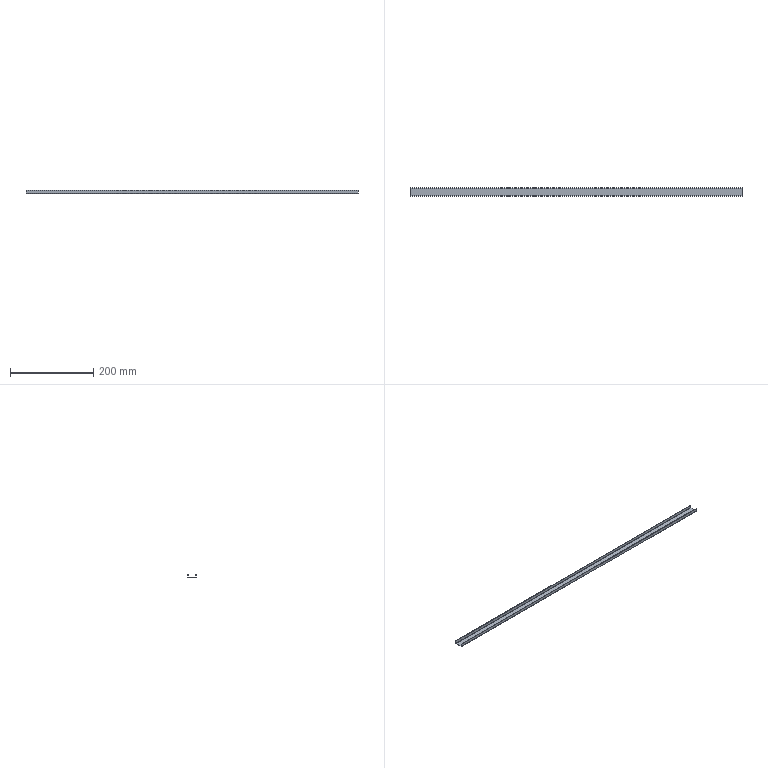Component | SolidWorks | AirFurnaceElectricalCabinet-DoorPanelAssembly-1_AirFurnaceElectricalCabinet-WireDuct-1 | 1 solid | 22 faces | volume 26513 mm3 | plane 18 | cylinder 4 | commonest cylinder face diameters 3 x2 1 x2